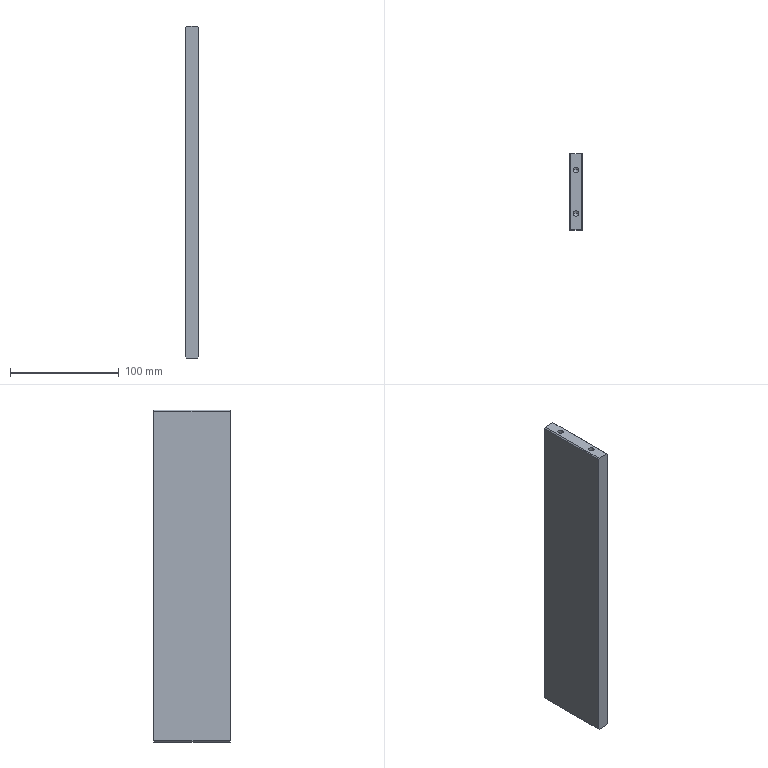Component | SolidWorks | Q1-A12-S21-Q1C.SLDASQ-1_Q1-A12-S21-Q1C-03A-1 | 1 solid | 26 faces | box 12 x 70 x 305 mm | volume 254843 mm3 | plane 10 | cylinder 8 | cone 8 | commonest cylinder face diameters 5 x8 | material Q235-Steel
build123d program:
from build123d import *

# Parameters (mm, degrees)
SKETCH1_W                 = 70
SKETCH1_H                 = 12
BOSS_EXTRUDE1_DEPTH       = 305
M6X1_0_TAPPED_HOLE1_D     = 5
M6X1_0_TAPPED_HOLE1_DEPTH = 15
M6X1_0_TAPPED_HOLE1_TIP   = 1.502
M6X1_0_TAPPED_HOLE2_D     = 5
M6X1_0_TAPPED_HOLE2_DEPTH = 15
M6X1_0_TAPPED_HOLE2_TIP   = 1.502
CHAMFER1_SIZE             = 1


with BuildPart() as part:
    # Sketch1 → Boss-Extrude1 (new body)
    with BuildSketch(Plane(origin=(0, 0, 0), x_dir=(1, 0, 0), z_dir=(0, 1, 0))):
        Rectangle(SKETCH1_W, SKETCH1_H)
    extrude(amount=BOSS_EXTRUDE1_DEPTH)

    # M6x1.0 Tapped Hole1
    with Locations(Plane(origin=(0, 305, 0), x_dir=(1, 0, 0), z_dir=(0, 1, 0))):
        with Locations((20, 0), (-20, 0)):
            Hole(M6X1_0_TAPPED_HOLE1_D / 2, depth=M6X1_0_TAPPED_HOLE1_DEPTH)
            with Locations((0, 0, -(M6X1_0_TAPPED_HOLE1_DEPTH + M6X1_0_TAPPED_HOLE1_TIP / 2))):  # 118° drill point
                Cone(0, M6X1_0_TAPPED_HOLE1_D / 2, M6X1_0_TAPPED_HOLE1_TIP, mode=Mode.SUBTRACT)

    # M6x1.0 Tapped Hole2
    with Locations(Plane(origin=(0, 0, 0), x_dir=(-1, 0, 0), z_dir=(0, -1, 0))):
        with Locations((20, 0), (-20, 0)):
            Hole(M6X1_0_TAPPED_HOLE2_D / 2, depth=M6X1_0_TAPPED_HOLE2_DEPTH)
            with Locations((0, 0, -(M6X1_0_TAPPED_HOLE2_DEPTH + M6X1_0_TAPPED_HOLE2_TIP / 2))):  # 118° drill point
                Cone(0, M6X1_0_TAPPED_HOLE2_D / 2, M6X1_0_TAPPED_HOLE2_TIP, mode=Mode.SUBTRACT)

    # Chamfer1
    chamfer1_edges = [part.edges().sort_by_distance(p)[0] for p in [
        (0, 305, 6),
        (0, 0, 6),
        (0, 0, -6),
        (0, 305, -6),
    ]]
    chamfer(chamfer1_edges, length=CHAMFER1_SIZE)


solid = part.part

# Placed as in the assembly
solid = solid.moved(Location((2095.5, 0, -152.5), (90, -90, 0)))
STEP:
#1=COLOUR_RGB('',0.7922,0.8196,0.9333);
#2=FILL_AREA_STYLE_COLOUR('',#1);
#3=FILL_AREA_STYLE('',(#2));
#4=SURFACE_STYLE_FILL_AREA(#3);
#5=SURFACE_SIDE_STYLE('',(#4));
#6=SURFACE_STYLE_USAGE(.BOTH.,#5);
#7=PRESENTATION_STYLE_ASSIGNMENT((#6));
#8=CARTESIAN_POINT('',(82.402,-0.7874,5.413));
#9=VERTEX_POINT('',#8);
#10=CARTESIAN_POINT('',(82.598,-0.7874,5.413));
#11=VERTEX_POINT('',#10);
#12=CARTESIAN_POINT('',(82.5,-0.7874,5.413));
#13=DIRECTION('',(0.,-0.,1.));
#14=DIRECTION('',(1.,0.,0.));
#15=AXIS2_PLACEMENT_3D('',#12,#13,#14);
#16=CIRCLE('',#15,0.09843);
#17=EDGE_CURVE('',#9,#11,#16,.T.);
#18=ORIENTED_EDGE('',*,*,#17,.F.);
#19=CARTESIAN_POINT('',(82.402,-0.7874,6.004));
#20=VERTEX_POINT('',#19);
#21=CARTESIAN_POINT('',(82.402,-0.7874,6.004));
#22=DIRECTION('',(0.,-0.,1.));
#23=VECTOR('',#22,39.37);
#24=LINE('',#21,#23);
#25=EDGE_CURVE('',#9,#20,#24,.T.);
#26=ORIENTED_EDGE('',*,*,#25,.T.);
#27=CARTESIAN_POINT('',(82.598,-0.7874,6.004));
#28=VERTEX_POINT('',#27);
#29=CARTESIAN_POINT('',(82.5,-0.7874,6.004));
#30=DIRECTION('',(0.,-0.,1.));
#31=DIRECTION('',(1.,0.,0.));
#32=AXIS2_PLACEMENT_3D('',#29,#30,#31);
#33=CIRCLE('',#32,0.09843);
#34=EDGE_CURVE('',#20,#28,#33,.T.);
#35=ORIENTED_EDGE('',*,*,#34,.T.);
#36=CARTESIAN_POINT('',(82.598,-0.7874,6.004));
#37=DIRECTION('',(0.,-0.,1.));
#38=VECTOR('',#37,39.37);
#39=LINE('',#36,#38);
#40=EDGE_CURVE('',#11,#28,#39,.T.);
#41=ORIENTED_EDGE('',*,*,#40,.F.);
#42=EDGE_LOOP('',(#18,#26,#35,#41));
#43=FACE_OUTER_BOUND('',#42,.T.);
#44=CARTESIAN_POINT('',(82.5,-0.7874,6.004));
#45=DIRECTION('',(0.,-0.,1.));
#46=DIRECTION('',(1.,0.,0.));
#47=AXIS2_PLACEMENT_3D('',#44,#45,#46);
#48=CYLINDRICAL_SURFACE('',#47,0.09843);
#49=ADVANCED_FACE('',(#43),#48,.F.);
#50=CARTESIAN_POINT('',(82.5,-0.7874,5.354));
#51=VERTEX_POINT('',#50);
#52=CARTESIAN_POINT('',(82.598,-0.7874,5.413));
#53=DIRECTION('',(0.8572,-0.,0.515));
#54=VECTOR('',#53,39.37);
#55=LINE('',#52,#54);
#56=EDGE_CURVE('',#51,#11,#55,.T.);
#57=ORIENTED_EDGE('',*,*,#56,.F.);
#58=CARTESIAN_POINT('',(82.402,-0.7874,5.413));
#59=DIRECTION('',(-0.8572,0.,0.515));
#60=VECTOR('',#59,39.37);
#61=LINE('',#58,#60);
#62=EDGE_CURVE('',#51,#9,#61,.T.);
#63=ORIENTED_EDGE('',*,*,#62,.T.);
#64=ORIENTED_EDGE('',*,*,#17,.T.);
#65=EDGE_LOOP('',(#57,#63,#64));
#66=FACE_OUTER_BOUND('',#65,.T.);
#67=CARTESIAN_POINT('',(82.5,-0.7874,5.413));
#68=DIRECTION('',(0.,-0.,1.));
#69=DIRECTION('',(1.,0.,0.));
#70=AXIS2_PLACEMENT_3D('',#67,#68,#69);
#71=CONICAL_SURFACE('',#70,0.09843,1.03);
#72=ADVANCED_FACE('',(#66),#71,.F.);
#73=CARTESIAN_POINT('',(82.402,0.7874,5.413));
#74=VERTEX_POINT('',#73);
#75=CARTESIAN_POINT('',(82.598,0.7874,5.413));
#76=VERTEX_POINT('',#75);
#77=CARTESIAN_POINT('',(82.5,0.7874,5.413));
#78=DIRECTION('',(0.,-0.,1.));
#79=DIRECTION('',(1.,0.,0.));
#80=AXIS2_PLACEMENT_3D('',#77,#78,#79);
#81=CIRCLE('',#80,0.09843);
#82=EDGE_CURVE('',#74,#76,#81,.T.);
#83=ORIENTED_EDGE('',*,*,#82,.F.);
#84=CARTESIAN_POINT('',(82.402,0.7874,6.004));
#85=VERTEX_POINT('',#84);
#86=CARTESIAN_POINT('',(82.402,0.7874,6.004));
#87=DIRECTION('',(0.,-0.,1.));
#88=VECTOR('',#87,39.37);
#89=LINE('',#86,#88);
#90=EDGE_CURVE('',#74,#85,#89,.T.);
#91=ORIENTED_EDGE('',*,*,#90,.T.);
#92=CARTESIAN_POINT('',(82.598,0.7874,6.004));
#93=VERTEX_POINT('',#92);
#94=CARTESIAN_POINT('',(82.5,0.7874,6.004));
#95=DIRECTION('',(0.,-0.,1.));
#96=DIRECTION('',(1.,0.,0.));
#97=AXIS2_PLACEMENT_3D('',#94,#95,#96);
#98=CIRCLE('',#97,0.09843);
#99=EDGE_CURVE('',#85,#93,#98,.T.);
#100=ORIENTED_EDGE('',*,*,#99,.T.);
#101=CARTESIAN_POINT('',(82.598,0.7874,6.004));
#102=DIRECTION('',(0.,-0.,1.));
#103=VECTOR('',#102,39.37);
#104=LINE('',#101,#103);
#105=EDGE_CURVE('',#76,#93,#104,.T.);
#106=ORIENTED_EDGE('',*,*,#105,.F.);
#107=EDGE_LOOP('',(#83,#91,#100,#106));
#108=FACE_OUTER_BOUND('',#107,.T.);
#109=CARTESIAN_POINT('',(82.5,0.7874,6.004));
#110=DIRECTION('',(0.,-0.,1.));
#111=DIRECTION('',(1.,0.,0.));
#112=AXIS2_PLACEMENT_3D('',#109,#110,#111);
#113=CYLINDRICAL_SURFACE('',#112,0.09843);
#114=ADVANCED_FACE('',(#108),#113,.F.);
#115=CARTESIAN_POINT('',(82.5,0.7874,5.354));
#116=VERTEX_POINT('',#115);
#117=CARTESIAN_POINT('',(82.598,0.7874,5.413));
#118=DIRECTION('',(0.8572,-0.,0.515));
#119=VECTOR('',#118,39.37);
#120=LINE('',#117,#119);
#121=EDGE_CURVE('',#116,#76,#120,.T.);
#122=ORIENTED_EDGE('',*,*,#121,.F.);
#123=CARTESIAN_POINT('',(82.402,0.7874,5.413));
#124=DIRECTION('',(-0.8572,0.,0.515));
#125=VECTOR('',#124,39.37);
#126=LINE('',#123,#125);
#127=EDGE_CURVE('',#116,#74,#126,.T.);
#128=ORIENTED_EDGE('',*,*,#127,.T.);
#129=ORIENTED_EDGE('',*,*,#82,.T.);
#130=EDGE_LOOP('',(#122,#128,#129));
#131=FACE_OUTER_BOUND('',#130,.T.);
#132=CARTESIAN_POINT('',(82.5,0.7874,5.413));
#133=DIRECTION('',(0.,-0.,1.));
#134=DIRECTION('',(1.,0.,0.));
#135=AXIS2_PLACEMENT_3D('',#132,#133,#134);
#136=CONICAL_SURFACE('',#135,0.09843,1.03);
#137=ADVANCED_FACE('',(#131),#136,.F.);
#138=CARTESIAN_POINT('',(82.598,0.7874,-5.413));
#139=VERTEX_POINT('',#138);
#140=CARTESIAN_POINT('',(82.402,0.7874,-5.413));
#141=VERTEX_POINT('',#140);
#142=CARTESIAN_POINT('',(82.5,0.7874,-5.413));
#143=DIRECTION('',(-0.,0.,-1.));
#144=DIRECTION('',(-1.,0.,0.));
#145=AXIS2_PLACEMENT_3D('',#142,#143,#144);
#146=CIRCLE('',#145,0.09843);
#147=EDGE_CURVE('',#139,#141,#146,.T.);
#148=ORIENTED_EDGE('',*,*,#147,.F.);
#149=CARTESIAN_POINT('',(82.598,0.7874,-6.004));
#150=VERTEX_POINT('',#149);
#151=CARTESIAN_POINT('',(82.598,0.7874,-6.004));
#152=DIRECTION('',(-0.,0.,-1.));
#153=VECTOR('',#152,39.37);
#154=LINE('',#151,#153);
#155=EDGE_CURVE('',#139,#150,#154,.T.);
#156=ORIENTED_EDGE('',*,*,#155,.T.);
#157=CARTESIAN_POINT('',(82.402,0.7874,-6.004));
#158=VERTEX_POINT('',#157);
#159=CARTESIAN_POINT('',(82.5,0.7874,-6.004));
#160=DIRECTION('',(-0.,0.,-1.));
#161=DIRECTION('',(-1.,0.,0.));
#162=AXIS2_PLACEMENT_3D('',#159,#160,#161);
#163=CIRCLE('',#162,0.09843);
#164=EDGE_CURVE('',#150,#158,#163,.T.);
#165=ORIENTED_EDGE('',*,*,#164,.T.);
#166=CARTESIAN_POINT('',(82.402,0.7874,-6.004));
#167=DIRECTION('',(-0.,0.,-1.));
#168=VECTOR('',#167,39.37);
#169=LINE('',#166,#168);
#170=EDGE_CURVE('',#141,#158,#169,.T.);
#171=ORIENTED_EDGE('',*,*,#170,.F.);
#172=EDGE_LOOP('',(#148,#156,#165,#171));
#173=FACE_OUTER_BOUND('',#172,.T.);
#174=CARTESIAN_POINT('',(82.5,0.7874,-6.004));
#175=DIRECTION('',(-0.,0.,-1.));
#176=DIRECTION('',(-1.,0.,0.));
#177=AXIS2_PLACEMENT_3D('',#174,#175,#176);
#178=CYLINDRICAL_SURFACE('',#177,0.09843);
#179=ADVANCED_FACE('',(#173),#178,.F.);
#180=CARTESIAN_POINT('',(82.5,0.7874,-5.354));
#181=VERTEX_POINT('',#180);
#182=CARTESIAN_POINT('',(82.402,0.7874,-5.413));
#183=DIRECTION('',(-0.8572,0.,-0.515));
#184=VECTOR('',#183,39.37);
#185=LINE('',#182,#184);
#186=EDGE_CURVE('',#181,#141,#185,.T.);
#187=ORIENTED_EDGE('',*,*,#186,.F.);
#188=CARTESIAN_POINT('',(82.598,0.7874,-5.413));
#189=DIRECTION('',(0.8572,0.,-0.515));
#190=VECTOR('',#189,39.37);
#191=LINE('',#188,#190);
#192=EDGE_CURVE('',#181,#139,#191,.T.);
#193=ORIENTED_EDGE('',*,*,#192,.T.);
#194=ORIENTED_EDGE('',*,*,#147,.T.);
#195=EDGE_LOOP('',(#187,#193,#194));
#196=FACE_OUTER_BOUND('',#195,.T.);
#197=CARTESIAN_POINT('',(82.5,0.7874,-5.413));
#198=DIRECTION('',(-0.,0.,-1.));
#199=DIRECTION('',(-1.,0.,0.));
#200=AXIS2_PLACEMENT_3D('',#197,#198,#199);
#201=CONICAL_SURFACE('',#200,0.09843,1.03);
#202=ADVANCED_FACE('',(#196),#201,.F.);
#203=CARTESIAN_POINT('',(82.598,-0.7874,-5.413));
#204=VERTEX_POINT('',#203);
#205=CARTESIAN_POINT('',(82.402,-0.7874,-5.413));
#206=VERTEX_POINT('',#205);
#207=CARTESIAN_POINT('',(82.5,-0.7874,-5.413));
#208=DIRECTION('',(-0.,0.,-1.));
#209=DIRECTION('',(-1.,0.,0.));
#210=AXIS2_PLACEMENT_3D('',#207,#208,#209);
#211=CIRCLE('',#210,0.09843);
#212=EDGE_CURVE('',#204,#206,#211,.T.);
#213=ORIENTED_EDGE('',*,*,#212,.F.);
#214=CARTESIAN_POINT('',(82.598,-0.7874,-6.004));
#215=VERTEX_POINT('',#214);
#216=CARTESIAN_POINT('',(82.598,-0.7874,-6.004));
#217=DIRECTION('',(-0.,0.,-1.));
#218=VECTOR('',#217,39.37);
#219=LINE('',#216,#218);
#220=EDGE_CURVE('',#204,#215,#219,.T.);
#221=ORIENTED_EDGE('',*,*,#220,.T.);
#222=CARTESIAN_POINT('',(82.402,-0.7874,-6.004));
#223=VERTEX_POINT('',#222);
#224=CARTESIAN_POINT('',(82.5,-0.7874,-6.004));
#225=DIRECTION('',(-0.,0.,-1.));
#226=DIRECTION('',(-1.,0.,0.));
#227=AXIS2_PLACEMENT_3D('',#224,#225,#226);
#228=CIRCLE('',#227,0.09843);
#229=EDGE_CURVE('',#215,#223,#228,.T.);
#230=ORIENTED_EDGE('',*,*,#229,.T.);
#231=CARTESIAN_POINT('',(82.402,-0.7874,-6.004));
#232=DIRECTION('',(-0.,0.,-1.));
#233=VECTOR('',#232,39.37);
#234=LINE('',#231,#233);
#235=EDGE_CURVE('',#206,#223,#234,.T.);
#236=ORIENTED_EDGE('',*,*,#235,.F.);
#237=EDGE_LOOP('',(#213,#221,#230,#236));
#238=FACE_OUTER_BOUND('',#237,.T.);
#239=CARTESIAN_POINT('',(82.5,-0.7874,-6.004));
#240=DIRECTION('',(-0.,0.,-1.));
#241=DIRECTION('',(-1.,0.,0.));
#242=AXIS2_PLACEMENT_3D('',#239,#240,#241);
#243=CYLINDRICAL_SURFACE('',#242,0.09843);
#244=ADVANCED_FACE('',(#238),#243,.F.);
#245=CARTESIAN_POINT('',(82.5,-0.7874,-5.354));
#246=VERTEX_POINT('',#245);
#247=CARTESIAN_POINT('',(82.402,-0.7874,-5.413));
#248=DIRECTION('',(-0.8572,0.,-0.515));
#249=VECTOR('',#248,39.37);
#250=LINE('',#247,#249);
#251=EDGE_CURVE('',#246,#206,#250,.T.);
#252=ORIENTED_EDGE('',*,*,#251,.F.);
#253=CARTESIAN_POINT('',(82.598,-0.7874,-5.413));
#254=DIRECTION('',(0.8572,0.,-0.515));
#255=VECTOR('',#254,39.37);
#256=LINE('',#253,#255);
#257=EDGE_CURVE('',#246,#204,#256,.T.);
#258=ORIENTED_EDGE('',*,*,#257,.T.);
#259=ORIENTED_EDGE('',*,*,#212,.T.);
#260=EDGE_LOOP('',(#252,#258,#259));
#261=FACE_OUTER_BOUND('',#260,.T.);
#262=CARTESIAN_POINT('',(82.5,-0.7874,-5.413));
#263=DIRECTION('',(-0.,0.,-1.));
#264=DIRECTION('',(-1.,0.,0.));
#265=AXIS2_PLACEMENT_3D('',#262,#263,#264);
#266=CONICAL_SURFACE('',#265,0.09843,1.03);
#267=ADVANCED_FACE('',(#261),#266,.F.);
#268=CARTESIAN_POINT('',(82.264,1.378,-5.965));
#269=VERTEX_POINT('',#268);
#270=CARTESIAN_POINT('',(82.264,1.378,5.965));
#271=VERTEX_POINT('',#270);
#272=CARTESIAN_POINT('',(82.264,1.378,-6.004));
#273=DIRECTION('',(0.,-0.,1.));
#274=VECTOR('',#273,39.37);
#275=LINE('',#272,#274);
#276=EDGE_CURVE('',#269,#271,#275,.T.);
#277=ORIENTED_EDGE('',*,*,#276,.T.);
#278=CARTESIAN_POINT('',(82.303,1.378,6.004));
#279=VERTEX_POINT('',#278);
#280=CARTESIAN_POINT('',(82.264,1.378,5.965));
#281=DIRECTION('',(0.7071,-0.,0.7071));
#282=VECTOR('',#281,39.37);
#283=LINE('',#280,#282);
#284=EDGE_CURVE('',#271,#279,#283,.T.);
#285=ORIENTED_EDGE('',*,*,#284,.T.);
#286=CARTESIAN_POINT('',(82.697,1.378,6.004));
#287=VERTEX_POINT('',#286);
#288=CARTESIAN_POINT('',(82.264,1.378,6.004));
#289=DIRECTION('',(1.,-0.,0.));
#290=VECTOR('',#289,39.37);
#291=LINE('',#288,#290);
#292=EDGE_CURVE('',#279,#287,#291,.T.);
#293=ORIENTED_EDGE('',*,*,#292,.T.);
#294=CARTESIAN_POINT('',(82.736,1.378,5.965));
#295=VERTEX_POINT('',#294);
#296=CARTESIAN_POINT('',(82.736,1.378,5.965));
#297=DIRECTION('',(0.7071,0.,-0.7071));
#298=VECTOR('',#297,39.37);
#299=LINE('',#296,#298);
#300=EDGE_CURVE('',#287,#295,#299,.T.);
#301=ORIENTED_EDGE('',*,*,#300,.T.);
#302=CARTESIAN_POINT('',(82.736,1.378,-5.965));
#303=VERTEX_POINT('',#302);
#304=CARTESIAN_POINT('',(82.736,1.378,-6.004));
#305=DIRECTION('',(0.,-0.,1.));
#306=VECTOR('',#305,39.37);
#307=LINE('',#304,#306);
#308=EDGE_CURVE('',#303,#295,#307,.T.);
#309=ORIENTED_EDGE('',*,*,#308,.F.);
#310=CARTESIAN_POINT('',(82.697,1.378,-6.004));
#311=VERTEX_POINT('',#310);
#312=CARTESIAN_POINT('',(82.697,1.378,-6.004));
#313=DIRECTION('',(-0.7071,0.,-0.7071));
#314=VECTOR('',#313,39.37);
#315=LINE('',#312,#314);
#316=EDGE_CURVE('',#303,#311,#315,.T.);
#317=ORIENTED_EDGE('',*,*,#316,.T.);
#318=CARTESIAN_POINT('',(82.303,1.378,-6.004));
#319=VERTEX_POINT('',#318);
#320=CARTESIAN_POINT('',(82.264,1.378,-6.004));
#321=DIRECTION('',(1.,-0.,0.));
#322=VECTOR('',#321,39.37);
#323=LINE('',#320,#322);
#324=EDGE_CURVE('',#319,#311,#323,.T.);
#325=ORIENTED_EDGE('',*,*,#324,.F.);
#326=CARTESIAN_POINT('',(82.303,1.378,-6.004));
#327=DIRECTION('',(-0.7071,-0.,0.7071));
#328=VECTOR('',#327,39.37);
#329=LINE('',#326,#328);
#330=EDGE_CURVE('',#319,#269,#329,.T.);
#331=ORIENTED_EDGE('',*,*,#330,.T.);
#332=EDGE_LOOP('',(#277,#285,#293,#301,#309,#317,#325,#331));
#333=FACE_OUTER_BOUND('',#332,.T.);
#334=CARTESIAN_POINT('',(82.264,1.378,-6.004));
#335=DIRECTION('',(-0.,-1.,-0.));
#336=DIRECTION('',(-1.,0.,-0.));
#337=AXIS2_PLACEMENT_3D('',#334,#335,#336);
#338=PLANE('',#337);
#339=ADVANCED_FACE('',(#333),#338,.F.);
#340=ORIENTED_EDGE('',*,*,#308,.T.);
#341=CARTESIAN_POINT('',(82.736,-1.378,5.965));
#342=VERTEX_POINT('',#341);
#343=CARTESIAN_POINT('',(82.736,-1.378,5.965));
#344=DIRECTION('',(-0.,-1.,-0.));
#345=VECTOR('',#344,39.37);
#346=LINE('',#343,#345);
#347=EDGE_CURVE('',#295,#342,#346,.T.);
#348=ORIENTED_EDGE('',*,*,#347,.T.);
#349=CARTESIAN_POINT('',(82.736,-1.378,-5.965));
#350=VERTEX_POINT('',#349);
#351=CARTESIAN_POINT('',(82.736,-1.378,-6.004));
#352=DIRECTION('',(0.,-0.,1.));
#353=VECTOR('',#352,39.37);
#354=LINE('',#351,#353);
#355=EDGE_CURVE('',#350,#342,#354,.T.);
#356=ORIENTED_EDGE('',*,*,#355,.F.);
#357=CARTESIAN_POINT('',(82.736,-1.378,-5.965));
#358=DIRECTION('',(0.,1.,0.));
#359=VECTOR('',#358,39.37);
#360=LINE('',#357,#359);
#361=EDGE_CURVE('',#350,#303,#360,.T.);
#362=ORIENTED_EDGE('',*,*,#361,.T.);
#363=EDGE_LOOP('',(#340,#348,#356,#362));
#364=FACE_OUTER_BOUND('',#363,.T.);
#365=CARTESIAN_POINT('',(82.736,-1.378,-6.004));
#366=DIRECTION('',(-1.,0.,-0.));
#367=DIRECTION('',(0.,1.,0.));
#368=AXIS2_PLACEMENT_3D('',#365,#366,#367);
#369=PLANE('',#368);
#370=ADVANCED_FACE('',(#364),#369,.F.);
#371=CARTESIAN_POINT('',(82.697,-1.378,6.004));
#372=VERTEX_POINT('',#371);
#373=CARTESIAN_POINT('',(82.303,-1.378,6.004));
#374=VERTEX_POINT('',#373);
#375=CARTESIAN_POINT('',(82.264,-1.378,6.004));
#376=DIRECTION('',(-1.,0.,-0.));
#377=VECTOR('',#376,39.37);
#378=LINE('',#375,#377);
#379=EDGE_CURVE('',#372,#374,#378,.T.);
#380=ORIENTED_EDGE('',*,*,#379,.T.);
#381=CARTESIAN_POINT('',(82.264,-1.378,5.965));
#382=VERTEX_POINT('',#381);
#383=CARTESIAN_POINT('',(82.264,-1.378,5.965));
#384=DIRECTION('',(-0.7071,0.,-0.7071));
#385=VECTOR('',#384,39.37);
#386=LINE('',#383,#385);
#387=EDGE_CURVE('',#374,#382,#386,.T.);
#388=ORIENTED_EDGE('',*,*,#387,.T.);
#389=CARTESIAN_POINT('',(82.264,-1.378,-5.965));
#390=VERTEX_POINT('',#389);
#391=CARTESIAN_POINT('',(82.264,-1.378,-6.004));
#392=DIRECTION('',(0.,-0.,1.));
#393=VECTOR('',#392,39.37);
#394=LINE('',#391,#393);
#395=EDGE_CURVE('',#390,#382,#394,.T.);
#396=ORIENTED_EDGE('',*,*,#395,.F.);
#397=CARTESIAN_POINT('',(82.303,-1.378,-6.004));
#398=VERTEX_POINT('',#397);
#399=CARTESIAN_POINT('',(82.303,-1.378,-6.004));
#400=DIRECTION('',(0.7071,0.,-0.7071));
#401=VECTOR('',#400,39.37);
#402=LINE('',#399,#401);
#403=EDGE_CURVE('',#390,#398,#402,.T.);
#404=ORIENTED_EDGE('',*,*,#403,.T.);
#405=CARTESIAN_POINT('',(82.697,-1.378,-6.004));
#406=VERTEX_POINT('',#405);
#407=CARTESIAN_POINT('',(82.264,-1.378,-6.004));
#408=DIRECTION('',(-1.,0.,-0.));
#409=VECTOR('',#408,39.37);
#410=LINE('',#407,#409);
#411=EDGE_CURVE('',#406,#398,#410,.T.);
#412=ORIENTED_EDGE('',*,*,#411,.F.);
#413=CARTESIAN_POINT('',(82.697,-1.378,-6.004));
#414=DIRECTION('',(0.7071,-0.,0.7071));
#415=VECTOR('',#414,39.37);
#416=LINE('',#413,#415);
#417=EDGE_CURVE('',#406,#350,#416,.T.);
#418=ORIENTED_EDGE('',*,*,#417,.T.);
#419=ORIENTED_EDGE('',*,*,#355,.T.);
#420=CARTESIAN_POINT('',(82.736,-1.378,5.965));
#421=DIRECTION('',(-0.7071,-0.,0.7071));
#422=VECTOR('',#421,39.37);
#423=LINE('',#420,#422);
#424=EDGE_CURVE('',#342,#372,#423,.T.);
#425=ORIENTED_EDGE('',*,*,#424,.T.);
#426=EDGE_LOOP('',(#380,#388,#396,#404,#412,#418,#419,#425));
#427=FACE_OUTER_BOUND('',#426,.T.);
#428=CARTESIAN_POINT('',(82.264,-1.378,-6.004));
#429=DIRECTION('',(0.,1.,0.));
#430=DIRECTION('',(1.,-0.,0.));
#431=AXIS2_PLACEMENT_3D('',#428,#429,#430);
#432=PLANE('',#431);
#433=ADVANCED_FACE('',(#427),#432,.F.);
#434=ORIENTED_EDGE('',*,*,#395,.T.);
#435=CARTESIAN_POINT('',(82.264,1.378,5.965));
#436=DIRECTION('',(0.,1.,0.));
#437=VECTOR('',#436,39.37);
#438=LINE('',#435,#437);
#439=EDGE_CURVE('',#382,#271,#438,.T.);
#440=ORIENTED_EDGE('',*,*,#439,.T.);
#441=ORIENTED_EDGE('',*,*,#276,.F.);
#442=CARTESIAN_POINT('',(82.264,-1.378,-5.965));
#443=DIRECTION('',(-0.,-1.,-0.));
#444=VECTOR('',#443,39.37);
#445=LINE('',#442,#444);
#446=EDGE_CURVE('',#269,#390,#445,.T.);
#447=ORIENTED_EDGE('',*,*,#446,.T.);
#448=EDGE_LOOP('',(#434,#440,#441,#447));
#449=FACE_OUTER_BOUND('',#448,.T.);
#450=CARTESIAN_POINT('',(82.264,-1.378,-6.004));
#451=DIRECTION('',(1.,-0.,0.));
#452=DIRECTION('',(-0.,-1.,-0.));
#453=AXIS2_PLACEMENT_3D('',#450,#451,#452);
#454=PLANE('',#453);
#455=ADVANCED_FACE('',(#449),#454,.F.);
#456=CARTESIAN_POINT('',(82.5,0.7874,-6.004));
#457=DIRECTION('',(-0.,0.,-1.));
#458=DIRECTION('',(-1.,0.,0.));
#459=AXIS2_PLACEMENT_3D('',#456,#457,#458);
#460=CIRCLE('',#459,0.09843);
#461=EDGE_CURVE('',#158,#150,#460,.T.);
#462=ORIENTED_EDGE('',*,*,#461,.F.);
#463=ORIENTED_EDGE('',*,*,#164,.F.);
#464=EDGE_LOOP('',(#462,#463));
#465=FACE_BOUND('',#464,.T.);
#466=CARTESIAN_POINT('',(82.5,-0.7874,-6.004));
#467=DIRECTION('',(-0.,0.,-1.));
#468=DIRECTION('',(-1.,0.,0.));
#469=AXIS2_PLACEMENT_3D('',#466,#467,#468);
#470=CIRCLE('',#469,0.09843);
#471=EDGE_CURVE('',#223,#215,#470,.T.);
#472=ORIENTED_EDGE('',*,*,#471,.F.);
#473=ORIENTED_EDGE('',*,*,#229,.F.);
#474=EDGE_LOOP('',(#472,#473));
#475=FACE_BOUND('',#474,.T.);
#476=ORIENTED_EDGE('',*,*,#324,.T.);
#477=CARTESIAN_POINT('',(82.697,0.,-6.004));
#478=DIRECTION('',(-0.,-1.,-0.));
#479=VECTOR('',#478,39.37);
#480=LINE('',#477,#479);
#481=EDGE_CURVE('',#311,#406,#480,.T.);
#482=ORIENTED_EDGE('',*,*,#481,.T.);
#483=ORIENTED_EDGE('',*,*,#411,.T.);
#484=CARTESIAN_POINT('',(82.303,0.,-6.004));
#485=DIRECTION('',(0.,1.,0.));
#486=VECTOR('',#485,39.37);
#487=LINE('',#484,#486);
#488=EDGE_CURVE('',#398,#319,#487,.T.);
#489=ORIENTED_EDGE('',*,*,#488,.T.);
#490=EDGE_LOOP('',(#476,#482,#483,#489));
#491=FACE_OUTER_BOUND('',#490,.T.);
#492=CARTESIAN_POINT('',(82.5,0.,-6.004));
#493=DIRECTION('',(-0.,-0.,1.));
#494=DIRECTION('',(1.,-0.,0.));
#495=AXIS2_PLACEMENT_3D('',#492,#493,#494);
#496=PLANE('',#495);
#497=ADVANCED_FACE('',(#465,#475,#491),#496,.F.);
#498=CARTESIAN_POINT('',(82.5,-0.7874,6.004));
#499=DIRECTION('',(0.,-0.,1.));
#500=DIRECTION('',(1.,0.,0.));
#501=AXIS2_PLACEMENT_3D('',#498,#499,#500);
#502=CIRCLE('',#501,0.09843);
#503=EDGE_CURVE('',#28,#20,#502,.T.);
#504=ORIENTED_EDGE('',*,*,#503,.F.);
#505=ORIENTED_EDGE('',*,*,#34,.F.);
#506=EDGE_LOOP('',(#504,#505));
#507=FACE_BOUND('',#506,.T.);
#508=CARTESIAN_POINT('',(82.5,0.7874,6.004));
#509=DIRECTION('',(0.,-0.,1.));
#510=DIRECTION('',(1.,0.,0.));
#511=AXIS2_PLACEMENT_3D('',#508,#509,#510);
#512=CIRCLE('',#511,0.09843);
#513=EDGE_CURVE('',#93,#85,#512,.T.);
#514=ORIENTED_EDGE('',*,*,#513,.F.);
#515=ORIENTED_EDGE('',*,*,#99,.F.);
#516=EDGE_LOOP('',(#514,#515));
#517=FACE_BOUND('',#516,.T.);
#518=ORIENTED_EDGE('',*,*,#292,.F.);
#519=CARTESIAN_POINT('',(82.303,-1.378,6.004));
#520=DIRECTION('',(-0.,-1.,-0.));
#521=VECTOR('',#520,39.37);
#522=LINE('',#519,#521);
#523=EDGE_CURVE('',#279,#374,#522,.T.);
#524=ORIENTED_EDGE('',*,*,#523,.T.);
#525=ORIENTED_EDGE('',*,*,#379,.F.);
#526=CARTESIAN_POINT('',(82.697,1.378,6.004));
#527=DIRECTION('',(0.,1.,0.));
#528=VECTOR('',#527,39.37);
#529=LINE('',#526,#528);
#530=EDGE_CURVE('',#372,#287,#529,.T.);
#531=ORIENTED_EDGE('',*,*,#530,.T.);
#532=EDGE_LOOP('',(#518,#524,#525,#531));
#533=FACE_OUTER_BOUND('',#532,.T.);
#534=CARTESIAN_POINT('',(82.5,-0.,6.004));
#535=DIRECTION('',(-0.,-0.,1.));
#536=DIRECTION('',(1.,-0.,0.));
#537=AXIS2_PLACEMENT_3D('',#534,#535,#536);
#538=PLANE('',#537);
#539=ADVANCED_FACE('',(#507,#517,#533),#538,.T.);
#540=ORIENTED_EDGE('',*,*,#257,.F.);
#541=ORIENTED_EDGE('',*,*,#251,.T.);
#542=CARTESIAN_POINT('',(82.5,-0.7874,-5.413));
#543=DIRECTION('',(-0.,0.,-1.));
#544=DIRECTION('',(-1.,0.,0.));
#545=AXIS2_PLACEMENT_3D('',#542,#543,#544);
#546=CIRCLE('',#545,0.09843);
#547=EDGE_CURVE('',#206,#204,#546,.T.);
#548=ORIENTED_EDGE('',*,*,#547,.T.);
#549=EDGE_LOOP('',(#540,#541,#548));
#550=FACE_OUTER_BOUND('',#549,.T.);
#551=CARTESIAN_POINT('',(82.5,-0.7874,-5.413));
#552=DIRECTION('',(-0.,0.,-1.));
#553=DIRECTION('',(-1.,0.,0.));
#554=AXIS2_PLACEMENT_3D('',#551,#552,#553);
#555=CONICAL_SURFACE('',#554,0.09843,1.03);
#556=ADVANCED_FACE('',(#550),#555,.F.);
#557=ORIENTED_EDGE('',*,*,#220,.F.);
#558=ORIENTED_EDGE('',*,*,#547,.F.);
#559=ORIENTED_EDGE('',*,*,#235,.T.);
#560=ORIENTED_EDGE('',*,*,#471,.T.);
#561=EDGE_LOOP('',(#557,#558,#559,#560));
#562=FACE_OUTER_BOUND('',#561,.T.);
#563=CARTESIAN_POINT('',(82.5,-0.7874,-6.004));
#564=DIRECTION('',(-0.,0.,-1.));
#565=DIRECTION('',(-1.,0.,0.));
#566=AXIS2_PLACEMENT_3D('',#563,#564,#565);
#567=CYLINDRICAL_SURFACE('',#566,0.09843);
#568=ADVANCED_FACE('',(#562),#567,.F.);
#569=ORIENTED_EDGE('',*,*,#192,.F.);
#570=ORIENTED_EDGE('',*,*,#186,.T.);
#571=CARTESIAN_POINT('',(82.5,0.7874,-5.413));
#572=DIRECTION('',(-0.,0.,-1.));
#573=DIRECTION('',(-1.,0.,0.));
#574=AXIS2_PLACEMENT_3D('',#571,#572,#573);
#575=CIRCLE('',#574,0.09843);
#576=EDGE_CURVE('',#141,#139,#575,.T.);
#577=ORIENTED_EDGE('',*,*,#576,.T.);
#578=EDGE_LOOP('',(#569,#570,#577));
#579=FACE_OUTER_BOUND('',#578,.T.);
#580=CARTESIAN_POINT('',(82.5,0.7874,-5.413));
#581=DIRECTION('',(-0.,0.,-1.));
#582=DIRECTION('',(-1.,0.,0.));
#583=AXIS2_PLACEMENT_3D('',#580,#581,#582);
#584=CONICAL_SURFACE('',#583,0.09843,1.03);
#585=ADVANCED_FACE('',(#579),#584,.F.);
#586=ORIENTED_EDGE('',*,*,#155,.F.);
#587=ORIENTED_EDGE('',*,*,#576,.F.);
#588=ORIENTED_EDGE('',*,*,#170,.T.);
#589=ORIENTED_EDGE('',*,*,#461,.T.);
#590=EDGE_LOOP('',(#586,#587,#588,#589));
#591=FACE_OUTER_BOUND('',#590,.T.);
#592=CARTESIAN_POINT('',(82.5,0.7874,-6.004));
#593=DIRECTION('',(-0.,0.,-1.));
#594=DIRECTION('',(-1.,0.,0.));
#595=AXIS2_PLACEMENT_3D('',#592,#593,#594);
#596=CYLINDRICAL_SURFACE('',#595,0.09843);
#597=ADVANCED_FACE('',(#591),#596,.F.);
#598=ORIENTED_EDGE('',*,*,#127,.F.);
#599=ORIENTED_EDGE('',*,*,#121,.T.);
#600=CARTESIAN_POINT('',(82.5,0.7874,5.413));
#601=DIRECTION('',(0.,-0.,1.));
#602=DIRECTION('',(1.,0.,0.));
#603=AXIS2_PLACEMENT_3D('',#600,#601,#602);
#604=CIRCLE('',#603,0.09843);
#605=EDGE_CURVE('',#76,#74,#604,.T.);
#606=ORIENTED_EDGE('',*,*,#605,.T.);
#607=EDGE_LOOP('',(#598,#599,#606));
#608=FACE_OUTER_BOUND('',#607,.T.);
#609=CARTESIAN_POINT('',(82.5,0.7874,5.413));
#610=DIRECTION('',(0.,-0.,1.));
#611=DIRECTION('',(1.,0.,0.));
#612=AXIS2_PLACEMENT_3D('',#609,#610,#611);
#613=CONICAL_SURFACE('',#612,0.09843,1.03);
#614=ADVANCED_FACE('',(#608),#613,.F.);
#615=ORIENTED_EDGE('',*,*,#90,.F.);
#616=ORIENTED_EDGE('',*,*,#605,.F.);
#617=ORIENTED_EDGE('',*,*,#105,.T.);
#618=ORIENTED_EDGE('',*,*,#513,.T.);
#619=EDGE_LOOP('',(#615,#616,#617,#618));
#620=FACE_OUTER_BOUND('',#619,.T.);
#621=CARTESIAN_POINT('',(82.5,0.7874,6.004));
#622=DIRECTION('',(0.,-0.,1.));
#623=DIRECTION('',(1.,0.,0.));
#624=AXIS2_PLACEMENT_3D('',#621,#622,#623);
#625=CYLINDRICAL_SURFACE('',#624,0.09843);
#626=ADVANCED_FACE('',(#620),#625,.F.);
#627=ORIENTED_EDGE('',*,*,#62,.F.);
#628=ORIENTED_EDGE('',*,*,#56,.T.);
#629=CARTESIAN_POINT('',(82.5,-0.7874,5.413));
#630=DIRECTION('',(0.,-0.,1.));
#631=DIRECTION('',(1.,0.,0.));
#632=AXIS2_PLACEMENT_3D('',#629,#630,#631);
#633=CIRCLE('',#632,0.09843);
#634=EDGE_CURVE('',#11,#9,#633,.T.);
#635=ORIENTED_EDGE('',*,*,#634,.T.);
#636=EDGE_LOOP('',(#627,#628,#635));
#637=FACE_OUTER_BOUND('',#636,.T.);
#638=CARTESIAN_POINT('',(82.5,-0.7874,5.413));
#639=DIRECTION('',(0.,-0.,1.));
#640=DIRECTION('',(1.,0.,0.));
#641=AXIS2_PLACEMENT_3D('',#638,#639,#640);
#642=CONICAL_SURFACE('',#641,0.09843,1.03);
#643=ADVANCED_FACE('',(#637),#642,.F.);
#644=ORIENTED_EDGE('',*,*,#25,.F.);
#645=ORIENTED_EDGE('',*,*,#634,.F.);
#646=ORIENTED_EDGE('',*,*,#40,.T.);
#647=ORIENTED_EDGE('',*,*,#503,.T.);
#648=EDGE_LOOP('',(#644,#645,#646,#647));
#649=FACE_OUTER_BOUND('',#648,.T.);
#650=CARTESIAN_POINT('',(82.5,-0.7874,6.004));
#651=DIRECTION('',(0.,-0.,1.));
#652=DIRECTION('',(1.,0.,0.));
#653=AXIS2_PLACEMENT_3D('',#650,#651,#652);
#654=CYLINDRICAL_SURFACE('',#653,0.09843);
#655=ADVANCED_FACE('',(#649),#654,.F.);
#656=ORIENTED_EDGE('',*,*,#387,.F.);
#657=ORIENTED_EDGE('',*,*,#523,.F.);
#658=ORIENTED_EDGE('',*,*,#284,.F.);
#659=ORIENTED_EDGE('',*,*,#439,.F.);
#660=EDGE_LOOP('',(#656,#657,#658,#659));
#661=FACE_OUTER_BOUND('',#660,.T.);
#662=CARTESIAN_POINT('',(82.264,-1.378,5.965));
#663=DIRECTION('',(-0.7071,-0.,0.7071));
#664=DIRECTION('',(-0.,-1.,-0.));
#665=AXIS2_PLACEMENT_3D('',#662,#663,#664);
#666=PLANE('',#665);
#667=ADVANCED_FACE('',(#661),#666,.T.);
#668=ORIENTED_EDGE('',*,*,#300,.F.);
#669=ORIENTED_EDGE('',*,*,#530,.F.);
#670=ORIENTED_EDGE('',*,*,#424,.F.);
#671=ORIENTED_EDGE('',*,*,#347,.F.);
#672=EDGE_LOOP('',(#668,#669,#670,#671));
#673=FACE_OUTER_BOUND('',#672,.T.);
#674=CARTESIAN_POINT('',(82.736,-1.378,5.965));
#675=DIRECTION('',(0.7071,-0.,0.7071));
#676=DIRECTION('',(0.,1.,0.));
#677=AXIS2_PLACEMENT_3D('',#674,#675,#676);
#678=PLANE('',#677);
#679=ADVANCED_FACE('',(#673),#678,.T.);
#680=ORIENTED_EDGE('',*,*,#316,.F.);
#681=ORIENTED_EDGE('',*,*,#361,.F.);
#682=ORIENTED_EDGE('',*,*,#417,.F.);
#683=ORIENTED_EDGE('',*,*,#481,.F.);
#684=EDGE_LOOP('',(#680,#681,#682,#683));
#685=FACE_OUTER_BOUND('',#684,.T.);
#686=CARTESIAN_POINT('',(82.697,0.,-6.004));
#687=DIRECTION('',(-0.7071,-0.,0.7071));
#688=DIRECTION('',(-0.,-1.,-0.));
#689=AXIS2_PLACEMENT_3D('',#686,#687,#688);
#690=PLANE('',#689);
#691=ADVANCED_FACE('',(#685),#690,.F.);
#692=ORIENTED_EDGE('',*,*,#403,.F.);
#693=ORIENTED_EDGE('',*,*,#446,.F.);
#694=ORIENTED_EDGE('',*,*,#330,.F.);
#695=ORIENTED_EDGE('',*,*,#488,.F.);
#696=EDGE_LOOP('',(#692,#693,#694,#695));
#697=FACE_OUTER_BOUND('',#696,.T.);
#698=CARTESIAN_POINT('',(82.303,0.,-6.004));
#699=DIRECTION('',(0.7071,-0.,0.7071));
#700=DIRECTION('',(0.,1.,0.));
#701=AXIS2_PLACEMENT_3D('',#698,#699,#700);
#702=PLANE('',#701);
#703=ADVANCED_FACE('',(#697),#702,.F.);
#704=CLOSED_SHELL('',(#49,#72,#114,#137,#179,#202,#244,#267,#339,#370,#433,#455,#497,#539,#556,#568,#585,#597,#614,#626,#643,#655,#667,#679,#691,#703));
#705=MANIFOLD_SOLID_BREP('',#704);
#706=STYLED_ITEM('',(#7),#705);
#707=(LENGTH_UNIT()NAMED_UNIT(*)SI_UNIT($,.METRE.));
#708=LENGTH_MEASURE_WITH_UNIT(LENGTH_MEASURE(0.0254),#707);
#709=DIMENSIONAL_EXPONENTS(1.,0.,0.,0.,0.,0.,0.);
#710=(CONVERSION_BASED_UNIT('',#708)LENGTH_UNIT()NAMED_UNIT(#709));
#711=UNCERTAINTY_MEASURE_WITH_UNIT(LENGTH_MEASURE(0.00001),#710,'','');
#712=(NAMED_UNIT(*)PLANE_ANGLE_UNIT()SI_UNIT($,.RADIAN.));
#713=(NAMED_UNIT(*)SI_UNIT($,.STERADIAN.)SOLID_ANGLE_UNIT());
#714=(GEOMETRIC_REPRESENTATION_CONTEXT(3)GLOBAL_UNCERTAINTY_ASSIGNED_CONTEXT((#711))GLOBAL_UNIT_ASSIGNED_CONTEXT((#710,#712,#713))REPRESENTATION_CONTEXT('',''));
#715=MECHANICAL_DESIGN_GEOMETRIC_PRESENTATION_REPRESENTATION('',(#706),#714);
#716=PRESENTATION_LAYER_ASSIGNMENT('','',(#706));
#717=CARTESIAN_POINT('',(0.,0.,0.));
#718=DIRECTION('',(0.,0.,1.));
#719=DIRECTION('',(1.,0.,0.));
#720=AXIS2_PLACEMENT_3D('',#717,#718,#719);
#721=(LENGTH_UNIT()NAMED_UNIT(*)SI_UNIT($,.METRE.));
#722=LENGTH_MEASURE_WITH_UNIT(LENGTH_MEASURE(0.0254),#721);
#723=DIMENSIONAL_EXPONENTS(1.,0.,0.,0.,0.,0.,0.);
#724=(CONVERSION_BASED_UNIT('',#722)LENGTH_UNIT()NAMED_UNIT(#723));
#725=UNCERTAINTY_MEASURE_WITH_UNIT(LENGTH_MEASURE(0.00001),#724,'','');
#726=(NAMED_UNIT(*)PLANE_ANGLE_UNIT()SI_UNIT($,.RADIAN.));
#727=(NAMED_UNIT(*)SI_UNIT($,.STERADIAN.)SOLID_ANGLE_UNIT());
#728=(GEOMETRIC_REPRESENTATION_CONTEXT(3)GLOBAL_UNCERTAINTY_ASSIGNED_CONTEXT((#725))GLOBAL_UNIT_ASSIGNED_CONTEXT((#724,#726,#727))REPRESENTATION_CONTEXT('',''));
#729=ADVANCED_BREP_SHAPE_REPRESENTATION('',(#705,#720),#728);